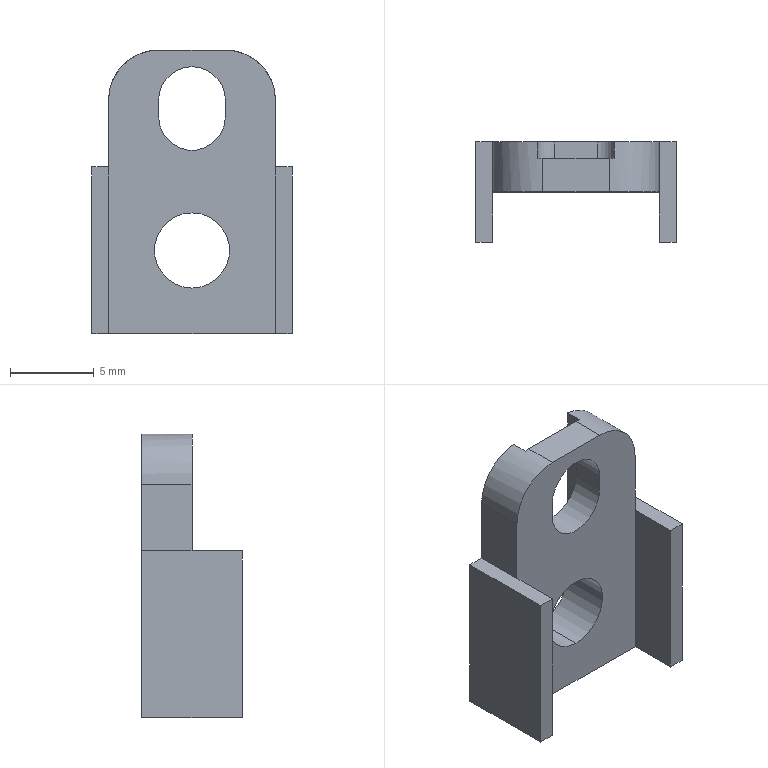Component | SolidWorks | BearingHousingAssembly-1_JawBuckleJaw2-1 | 1 solid | 29 faces | box 12 x 6 x 17 mm | volume 497 mm3 | plane 20 | cylinder 9 | commonest cylinder face diameters 4 x3 4.5 x2 6 x2 2 x2
build123d program:
from build123d import *

# Parameters (mm, degrees)
SKETCH1_W                  = 17
SKETCH1_H                  = 10
BOSS_EXTRUDE1_DEPTH        = 3
F_4_5_4_5_DIAMETER_HOLE1_D = 4.5
SKETCH4_W                  = 6
SKETCH4_H                  = 1
BOSS_EXTRUDE2_DEPTH        = 10
FILLET1_R                  = 3
CUT_EXTRUDE1_DEPTH         = 20
SKETCH6_W                  = 11.734
SKETCH6_H                  = 4.6
CUT_EXTRUDE2_DEPTH         = 1
FILLET2_R                  = 1


with BuildPart() as part:
    # Sketch1 → Boss-Extrude1 (new body)
    with BuildSketch(Plane.XY):
        with Locations((8.5, 0)):
            Rectangle(SKETCH1_W, SKETCH1_H)
    extrude(amount=BOSS_EXTRUDE1_DEPTH)

    # 4.5 _4.5_ Diameter Hole1 (through all)
    with Locations(Plane(origin=(0, 0, 0), x_dir=(-1, 0, 0), z_dir=(0, 0, -1))):
        with Locations((-5, 0)):
            Hole(F_4_5_4_5_DIAMETER_HOLE1_D / 2)

    # Sketch4 → Boss-Extrude2 (add)
    with BuildSketch(Plane.ZY):
        with Locations((0, 5.5)):
            Rectangle(SKETCH4_W, SKETCH4_H)
        with Locations((0, -5.5)):
            Rectangle(SKETCH4_W, SKETCH4_H)
    extrude(amount=-BOSS_EXTRUDE2_DEPTH)

    # Fillet1
    fillet1_edges = [part.edges().sort_by_distance(p)[0] for p in [
        (17, -5, 1.5),
        (17, 5, 1.5),
    ]]
    fillet(fillet1_edges, radius=FILLET1_R)

    # Sketch5 → Cut-Extrude1 (cut, through all)
    with BuildSketch(Plane.XY.offset(3)):
        with BuildLine():
            Line((13, 2), (14, 2))
            ThreePointArc((14, 2), (16, 0), (14, -2))
            Line((14, -2), (13, -2))
            ThreePointArc((13, -2), (11, 0), (13, 2))
        make_face()
    extrude(amount=-CUT_EXTRUDE1_DEPTH, mode=Mode.SUBTRACT)

    # Sketch6 → Cut-Extrude2 (cut)
    with BuildSketch(Plane.XY.offset(3)):
        with Locations((13.867, 0)):
            Rectangle(SKETCH6_W, SKETCH6_H)
    extrude(amount=-CUT_EXTRUDE2_DEPTH, mode=Mode.SUBTRACT)

    # Fillet2
    fillet2_edges = [part.edges().sort_by_distance(p)[0] for p in [
        (8, -2.3, 2.5),
        (8, 2.3, 2.5),
    ]]
    fillet(fillet2_edges, radius=FILLET2_R)


solid = part.part

# Placed as in the assembly
solid = solid.moved(Location((-38.666, 341.064, -6), (-90, 0, -90)))
STEP:
#1=CARTESIAN_POINT('',(-1.522,13.546,0.04921));
#2=VERTEX_POINT('',#1);
#3=CARTESIAN_POINT('',(-1.522,13.546,-0.128));
#4=VERTEX_POINT('',#3);
#5=CARTESIAN_POINT('',(-1.522,13.546,-0.03937));
#6=DIRECTION('',(-0.,-1.,0.));
#7=DIRECTION('',(-0.,0.,-1.));
#8=AXIS2_PLACEMENT_3D('',#5,#6,#7);
#9=CIRCLE('',#8,0.08858);
#10=EDGE_CURVE('',#2,#4,#9,.T.);
#11=ORIENTED_EDGE('',*,*,#10,.F.);
#12=CARTESIAN_POINT('',(-1.522,13.428,0.04921));
#13=VERTEX_POINT('',#12);
#14=CARTESIAN_POINT('',(-1.522,13.428,0.04921));
#15=DIRECTION('',(-0.,-1.,0.));
#16=VECTOR('',#15,39.37);
#17=LINE('',#14,#16);
#18=EDGE_CURVE('',#2,#13,#17,.T.);
#19=ORIENTED_EDGE('',*,*,#18,.T.);
#20=CARTESIAN_POINT('',(-1.522,13.428,-0.128));
#21=VERTEX_POINT('',#20);
#22=CARTESIAN_POINT('',(-1.522,13.428,-0.03937));
#23=DIRECTION('',(-0.,-1.,0.));
#24=DIRECTION('',(-0.,0.,-1.));
#25=AXIS2_PLACEMENT_3D('',#22,#23,#24);
#26=CIRCLE('',#25,0.08858);
#27=EDGE_CURVE('',#13,#21,#26,.T.);
#28=ORIENTED_EDGE('',*,*,#27,.T.);
#29=CARTESIAN_POINT('',(-1.522,13.428,-0.128));
#30=DIRECTION('',(-0.,-1.,0.));
#31=VECTOR('',#30,39.37);
#32=LINE('',#29,#31);
#33=EDGE_CURVE('',#4,#21,#32,.T.);
#34=ORIENTED_EDGE('',*,*,#33,.F.);
#35=EDGE_LOOP('',(#11,#19,#28,#34));
#36=FACE_OUTER_BOUND('',#35,.T.);
#37=CARTESIAN_POINT('',(-1.522,13.428,-0.03937));
#38=DIRECTION('',(-0.,-1.,0.));
#39=DIRECTION('',(-0.,0.,-1.));
#40=AXIS2_PLACEMENT_3D('',#37,#38,#39);
#41=CYLINDRICAL_SURFACE('',#40,0.08858);
#42=ADVANCED_FACE('',(#36),#41,.F.);
#43=CARTESIAN_POINT('',(-1.522,13.428,0.3937));
#44=VERTEX_POINT('',#43);
#45=CARTESIAN_POINT('',(-1.444,13.428,0.315));
#46=VERTEX_POINT('',#45);
#47=CARTESIAN_POINT('',(-1.522,13.428,0.315));
#48=DIRECTION('',(0.,1.,-0.));
#49=DIRECTION('',(0.,0.,1.));
#50=AXIS2_PLACEMENT_3D('',#47,#48,#49);
#51=CIRCLE('',#50,0.07874);
#52=EDGE_CURVE('',#44,#46,#51,.T.);
#53=ORIENTED_EDGE('',*,*,#52,.F.);
#54=CARTESIAN_POINT('',(-1.522,13.506,0.3937));
#55=VERTEX_POINT('',#54);
#56=CARTESIAN_POINT('',(-1.522,13.31,0.3937));
#57=DIRECTION('',(0.,1.,-0.));
#58=VECTOR('',#57,39.37);
#59=LINE('',#56,#58);
#60=EDGE_CURVE('',#44,#55,#59,.T.);
#61=ORIENTED_EDGE('',*,*,#60,.T.);
#62=CARTESIAN_POINT('',(-1.444,13.506,0.315));
#63=VERTEX_POINT('',#62);
#64=CARTESIAN_POINT('',(-1.522,13.506,0.315));
#65=DIRECTION('',(-0.,-1.,0.));
#66=DIRECTION('',(0.,0.,1.));
#67=AXIS2_PLACEMENT_3D('',#64,#65,#66);
#68=CIRCLE('',#67,0.07874);
#69=EDGE_CURVE('',#63,#55,#68,.T.);
#70=ORIENTED_EDGE('',*,*,#69,.F.);
#71=CARTESIAN_POINT('',(-1.444,13.31,0.315));
#72=DIRECTION('',(0.,1.,-0.));
#73=VECTOR('',#72,39.37);
#74=LINE('',#71,#73);
#75=EDGE_CURVE('',#46,#63,#74,.T.);
#76=ORIENTED_EDGE('',*,*,#75,.F.);
#77=EDGE_LOOP('',(#53,#61,#70,#76));
#78=FACE_OUTER_BOUND('',#77,.T.);
#79=CARTESIAN_POINT('',(-1.522,13.31,0.315));
#80=DIRECTION('',(0.,1.,-0.));
#81=DIRECTION('',(0.,0.,1.));
#82=AXIS2_PLACEMENT_3D('',#79,#80,#81);
#83=CYLINDRICAL_SURFACE('',#82,0.07874);
#84=ADVANCED_FACE('',(#78),#83,.F.);
#85=CARTESIAN_POINT('',(-1.601,13.506,0.4331));
#86=VERTEX_POINT('',#85);
#87=CARTESIAN_POINT('',(-1.444,13.506,0.4331));
#88=VERTEX_POINT('',#87);
#89=CARTESIAN_POINT('',(-1.325,13.506,0.4331));
#90=DIRECTION('',(1.,-0.,-0.));
#91=VECTOR('',#90,39.37);
#92=LINE('',#89,#91);
#93=EDGE_CURVE('',#86,#88,#92,.T.);
#94=ORIENTED_EDGE('',*,*,#93,.F.);
#95=CARTESIAN_POINT('',(-1.601,13.428,0.4331));
#96=VERTEX_POINT('',#95);
#97=CARTESIAN_POINT('',(-1.601,13.546,0.4331));
#98=DIRECTION('',(-0.,-1.,0.));
#99=VECTOR('',#98,39.37);
#100=LINE('',#97,#99);
#101=EDGE_CURVE('',#86,#96,#100,.T.);
#102=ORIENTED_EDGE('',*,*,#101,.T.);
#103=CARTESIAN_POINT('',(-1.444,13.428,0.4331));
#104=VERTEX_POINT('',#103);
#105=CARTESIAN_POINT('',(-1.325,13.428,0.4331));
#106=DIRECTION('',(1.,-0.,-0.));
#107=VECTOR('',#106,39.37);
#108=LINE('',#105,#107);
#109=EDGE_CURVE('',#96,#104,#108,.T.);
#110=ORIENTED_EDGE('',*,*,#109,.T.);
#111=CARTESIAN_POINT('',(-1.444,13.546,0.4331));
#112=DIRECTION('',(0.,1.,-0.));
#113=VECTOR('',#112,39.37);
#114=LINE('',#111,#113);
#115=EDGE_CURVE('',#104,#88,#114,.T.);
#116=ORIENTED_EDGE('',*,*,#115,.T.);
#117=EDGE_LOOP('',(#94,#102,#110,#116));
#118=FACE_OUTER_BOUND('',#117,.T.);
#119=CARTESIAN_POINT('',(-1.325,13.546,0.4331));
#120=DIRECTION('',(-0.,-0.,-1.));
#121=DIRECTION('',(0.,1.,-0.));
#122=AXIS2_PLACEMENT_3D('',#119,#120,#121);
#123=PLANE('',#122);
#124=ADVANCED_FACE('',(#118),#123,.F.);
#125=CARTESIAN_POINT('',(-1.601,13.506,0.2756));
#126=VERTEX_POINT('',#125);
#127=CARTESIAN_POINT('',(-1.444,13.506,0.2756));
#128=VERTEX_POINT('',#127);
#129=CARTESIAN_POINT('',(-1.522,13.506,0.2756));
#130=DIRECTION('',(-0.,-1.,0.));
#131=DIRECTION('',(0.,0.,1.));
#132=AXIS2_PLACEMENT_3D('',#129,#130,#131);
#133=CIRCLE('',#132,0.07874);
#134=EDGE_CURVE('',#126,#128,#133,.T.);
#135=ORIENTED_EDGE('',*,*,#134,.F.);
#136=CARTESIAN_POINT('',(-1.601,13.428,0.2756));
#137=VERTEX_POINT('',#136);
#138=CARTESIAN_POINT('',(-1.601,13.31,0.2756));
#139=DIRECTION('',(0.,1.,-0.));
#140=VECTOR('',#139,39.37);
#141=LINE('',#138,#140);
#142=EDGE_CURVE('',#137,#126,#141,.T.);
#143=ORIENTED_EDGE('',*,*,#142,.F.);
#144=CARTESIAN_POINT('',(-1.444,13.428,0.2756));
#145=VERTEX_POINT('',#144);
#146=CARTESIAN_POINT('',(-1.522,13.428,0.2756));
#147=DIRECTION('',(0.,1.,-0.));
#148=DIRECTION('',(0.,0.,1.));
#149=AXIS2_PLACEMENT_3D('',#146,#147,#148);
#150=CIRCLE('',#149,0.07874);
#151=EDGE_CURVE('',#145,#137,#150,.T.);
#152=ORIENTED_EDGE('',*,*,#151,.F.);
#153=CARTESIAN_POINT('',(-1.444,13.31,0.2756));
#154=DIRECTION('',(0.,1.,-0.));
#155=VECTOR('',#154,39.37);
#156=LINE('',#153,#155);
#157=EDGE_CURVE('',#145,#128,#156,.T.);
#158=ORIENTED_EDGE('',*,*,#157,.T.);
#159=EDGE_LOOP('',(#135,#143,#152,#158));
#160=FACE_OUTER_BOUND('',#159,.T.);
#161=CARTESIAN_POINT('',(-1.522,13.31,0.2756));
#162=DIRECTION('',(0.,1.,-0.));
#163=DIRECTION('',(0.,0.,1.));
#164=AXIS2_PLACEMENT_3D('',#161,#162,#163);
#165=CYLINDRICAL_SURFACE('',#164,0.07874);
#166=ADVANCED_FACE('',(#160),#165,.F.);
#167=CARTESIAN_POINT('',(-1.444,13.506,0.2756));
#168=DIRECTION('',(0.,0.,1.));
#169=VECTOR('',#168,39.37);
#170=LINE('',#167,#169);
#171=EDGE_CURVE('',#128,#63,#170,.T.);
#172=ORIENTED_EDGE('',*,*,#171,.F.);
#173=ORIENTED_EDGE('',*,*,#157,.F.);
#174=CARTESIAN_POINT('',(-1.444,13.428,-0.2362));
#175=DIRECTION('',(-0.,-0.,-1.));
#176=VECTOR('',#175,39.37);
#177=LINE('',#174,#176);
#178=EDGE_CURVE('',#46,#145,#177,.T.);
#179=ORIENTED_EDGE('',*,*,#178,.F.);
#180=ORIENTED_EDGE('',*,*,#75,.T.);
#181=EDGE_LOOP('',(#172,#173,#179,#180));
#182=FACE_OUTER_BOUND('',#181,.T.);
#183=CARTESIAN_POINT('',(-1.444,13.31,0.2756));
#184=DIRECTION('',(1.,-0.,-0.));
#185=DIRECTION('',(0.,1.,-0.));
#186=AXIS2_PLACEMENT_3D('',#183,#184,#185);
#187=PLANE('',#186);
#188=ADVANCED_FACE('',(#182),#187,.F.);
#189=ORIENTED_EDGE('',*,*,#60,.F.);
#190=CARTESIAN_POINT('',(-1.601,13.428,0.315));
#191=VERTEX_POINT('',#190);
#192=CARTESIAN_POINT('',(-1.522,13.428,0.315));
#193=DIRECTION('',(0.,1.,-0.));
#194=DIRECTION('',(0.,0.,1.));
#195=AXIS2_PLACEMENT_3D('',#192,#193,#194);
#196=CIRCLE('',#195,0.07874);
#197=EDGE_CURVE('',#191,#44,#196,.T.);
#198=ORIENTED_EDGE('',*,*,#197,.F.);
#199=CARTESIAN_POINT('',(-1.601,13.506,0.315));
#200=VERTEX_POINT('',#199);
#201=CARTESIAN_POINT('',(-1.601,13.31,0.315));
#202=DIRECTION('',(0.,1.,-0.));
#203=VECTOR('',#202,39.37);
#204=LINE('',#201,#203);
#205=EDGE_CURVE('',#191,#200,#204,.T.);
#206=ORIENTED_EDGE('',*,*,#205,.T.);
#207=CARTESIAN_POINT('',(-1.522,13.506,0.315));
#208=DIRECTION('',(-0.,-1.,0.));
#209=DIRECTION('',(0.,0.,1.));
#210=AXIS2_PLACEMENT_3D('',#207,#208,#209);
#211=CIRCLE('',#210,0.07874);
#212=EDGE_CURVE('',#55,#200,#211,.T.);
#213=ORIENTED_EDGE('',*,*,#212,.F.);
#214=EDGE_LOOP('',(#189,#198,#206,#213));
#215=FACE_OUTER_BOUND('',#214,.T.);
#216=CARTESIAN_POINT('',(-1.522,13.31,0.315));
#217=DIRECTION('',(0.,1.,-0.));
#218=DIRECTION('',(0.,0.,1.));
#219=AXIS2_PLACEMENT_3D('',#216,#217,#218);
#220=CYLINDRICAL_SURFACE('',#219,0.07874);
#221=ADVANCED_FACE('',(#215),#220,.F.);
#222=CARTESIAN_POINT('',(-1.601,13.506,0.2756));
#223=DIRECTION('',(-0.,-0.,-1.));
#224=VECTOR('',#223,39.37);
#225=LINE('',#222,#224);
#226=EDGE_CURVE('',#200,#126,#225,.T.);
#227=ORIENTED_EDGE('',*,*,#226,.F.);
#228=ORIENTED_EDGE('',*,*,#205,.F.);
#229=CARTESIAN_POINT('',(-1.601,13.428,-0.2362));
#230=DIRECTION('',(0.,0.,1.));
#231=VECTOR('',#230,39.37);
#232=LINE('',#229,#231);
#233=EDGE_CURVE('',#137,#191,#232,.T.);
#234=ORIENTED_EDGE('',*,*,#233,.F.);
#235=ORIENTED_EDGE('',*,*,#142,.T.);
#236=EDGE_LOOP('',(#227,#228,#234,#235));
#237=FACE_OUTER_BOUND('',#236,.T.);
#238=CARTESIAN_POINT('',(-1.601,13.31,0.2756));
#239=DIRECTION('',(-1.,0.,0.));
#240=DIRECTION('',(-0.,-1.,0.));
#241=AXIS2_PLACEMENT_3D('',#238,#239,#240);
#242=PLANE('',#241);
#243=ADVANCED_FACE('',(#237),#242,.F.);
#244=CARTESIAN_POINT('',(-1.325,13.428,-0.2362));
#245=VERTEX_POINT('',#244);
#246=CARTESIAN_POINT('',(-1.719,13.428,-0.2362));
#247=VERTEX_POINT('',#246);
#248=CARTESIAN_POINT('',(-1.325,13.428,-0.2362));
#249=DIRECTION('',(-1.,0.,0.));
#250=VECTOR('',#249,39.37);
#251=LINE('',#248,#250);
#252=EDGE_CURVE('',#245,#247,#251,.T.);
#253=ORIENTED_EDGE('',*,*,#252,.T.);
#254=CARTESIAN_POINT('',(-1.719,13.31,-0.2362));
#255=VERTEX_POINT('',#254);
#256=CARTESIAN_POINT('',(-1.719,13.546,-0.2362));
#257=DIRECTION('',(-0.,-1.,0.));
#258=VECTOR('',#257,39.37);
#259=LINE('',#256,#258);
#260=EDGE_CURVE('',#247,#255,#259,.T.);
#261=ORIENTED_EDGE('',*,*,#260,.T.);
#262=CARTESIAN_POINT('',(-1.758,13.31,-0.2362));
#263=VERTEX_POINT('',#262);
#264=CARTESIAN_POINT('',(-1.719,13.31,-0.2362));
#265=DIRECTION('',(-1.,0.,0.));
#266=VECTOR('',#265,39.37);
#267=LINE('',#264,#266);
#268=EDGE_CURVE('',#255,#263,#267,.T.);
#269=ORIENTED_EDGE('',*,*,#268,.T.);
#270=CARTESIAN_POINT('',(-1.758,13.546,-0.2362));
#271=VERTEX_POINT('',#270);
#272=CARTESIAN_POINT('',(-1.758,13.546,-0.2362));
#273=DIRECTION('',(0.,1.,-0.));
#274=VECTOR('',#273,39.37);
#275=LINE('',#272,#274);
#276=EDGE_CURVE('',#263,#271,#275,.T.);
#277=ORIENTED_EDGE('',*,*,#276,.T.);
#278=CARTESIAN_POINT('',(-1.286,13.546,-0.2362));
#279=VERTEX_POINT('',#278);
#280=CARTESIAN_POINT('',(-1.325,13.546,-0.2362));
#281=DIRECTION('',(-1.,0.,0.));
#282=VECTOR('',#281,39.37);
#283=LINE('',#280,#282);
#284=EDGE_CURVE('',#279,#271,#283,.T.);
#285=ORIENTED_EDGE('',*,*,#284,.F.);
#286=CARTESIAN_POINT('',(-1.286,13.31,-0.2362));
#287=VERTEX_POINT('',#286);
#288=CARTESIAN_POINT('',(-1.286,13.546,-0.2362));
#289=DIRECTION('',(-0.,-1.,0.));
#290=VECTOR('',#289,39.37);
#291=LINE('',#288,#290);
#292=EDGE_CURVE('',#279,#287,#291,.T.);
#293=ORIENTED_EDGE('',*,*,#292,.T.);
#294=CARTESIAN_POINT('',(-1.325,13.31,-0.2362));
#295=VERTEX_POINT('',#294);
#296=CARTESIAN_POINT('',(-1.325,13.31,-0.2362));
#297=DIRECTION('',(-1.,0.,0.));
#298=VECTOR('',#297,39.37);
#299=LINE('',#296,#298);
#300=EDGE_CURVE('',#287,#295,#299,.T.);
#301=ORIENTED_EDGE('',*,*,#300,.T.);
#302=CARTESIAN_POINT('',(-1.325,13.546,-0.2362));
#303=DIRECTION('',(0.,1.,-0.));
#304=VECTOR('',#303,39.37);
#305=LINE('',#302,#304);
#306=EDGE_CURVE('',#295,#245,#305,.T.);
#307=ORIENTED_EDGE('',*,*,#306,.T.);
#308=EDGE_LOOP('',(#253,#261,#269,#277,#285,#293,#301,#307));
#309=FACE_OUTER_BOUND('',#308,.T.);
#310=CARTESIAN_POINT('',(-1.325,13.546,-0.2362));
#311=DIRECTION('',(0.,0.,1.));
#312=DIRECTION('',(1.,-0.,-0.));
#313=AXIS2_PLACEMENT_3D('',#310,#311,#312);
#314=PLANE('',#313);
#315=ADVANCED_FACE('',(#309),#314,.F.);
#316=CARTESIAN_POINT('',(-1.719,13.428,0.1575));
#317=VERTEX_POINT('',#316);
#318=CARTESIAN_POINT('',(-1.719,13.428,0.315));
#319=VERTEX_POINT('',#318);
#320=CARTESIAN_POINT('',(-1.719,13.428,-0.2362));
#321=DIRECTION('',(0.,0.,1.));
#322=VECTOR('',#321,39.37);
#323=LINE('',#320,#322);
#324=EDGE_CURVE('',#317,#319,#323,.T.);
#325=ORIENTED_EDGE('',*,*,#324,.T.);
#326=CARTESIAN_POINT('',(-1.719,13.546,0.315));
#327=VERTEX_POINT('',#326);
#328=CARTESIAN_POINT('',(-1.719,13.546,0.315));
#329=DIRECTION('',(0.,1.,-0.));
#330=VECTOR('',#329,39.37);
#331=LINE('',#328,#330);
#332=EDGE_CURVE('',#319,#327,#331,.T.);
#333=ORIENTED_EDGE('',*,*,#332,.T.);
#334=CARTESIAN_POINT('',(-1.719,13.546,0.1575));
#335=VERTEX_POINT('',#334);
#336=CARTESIAN_POINT('',(-1.719,13.546,-0.2362));
#337=DIRECTION('',(0.,0.,1.));
#338=VECTOR('',#337,39.37);
#339=LINE('',#336,#338);
#340=EDGE_CURVE('',#335,#327,#339,.T.);
#341=ORIENTED_EDGE('',*,*,#340,.F.);
#342=CARTESIAN_POINT('',(-1.719,13.546,0.1575));
#343=DIRECTION('',(-0.,-1.,0.));
#344=VECTOR('',#343,39.37);
#345=LINE('',#342,#344);
#346=EDGE_CURVE('',#335,#317,#345,.T.);
#347=ORIENTED_EDGE('',*,*,#346,.T.);
#348=EDGE_LOOP('',(#325,#333,#341,#347));
#349=FACE_OUTER_BOUND('',#348,.T.);
#350=CARTESIAN_POINT('',(-1.719,13.546,-0.2362));
#351=DIRECTION('',(1.,-0.,-0.));
#352=DIRECTION('',(0.,1.,-0.));
#353=AXIS2_PLACEMENT_3D('',#350,#351,#352);
#354=PLANE('',#353);
#355=ADVANCED_FACE('',(#349),#354,.F.);
#356=CARTESIAN_POINT('',(-1.325,13.546,0.315));
#357=VERTEX_POINT('',#356);
#358=CARTESIAN_POINT('',(-1.325,13.546,0.1575));
#359=VERTEX_POINT('',#358);
#360=CARTESIAN_POINT('',(-1.325,13.546,-0.2362));
#361=DIRECTION('',(-0.,-0.,-1.));
#362=VECTOR('',#361,39.37);
#363=LINE('',#360,#362);
#364=EDGE_CURVE('',#357,#359,#363,.T.);
#365=ORIENTED_EDGE('',*,*,#364,.F.);
#366=CARTESIAN_POINT('',(-1.325,13.428,0.315));
#367=VERTEX_POINT('',#366);
#368=CARTESIAN_POINT('',(-1.325,13.546,0.315));
#369=DIRECTION('',(-0.,-1.,0.));
#370=VECTOR('',#369,39.37);
#371=LINE('',#368,#370);
#372=EDGE_CURVE('',#357,#367,#371,.T.);
#373=ORIENTED_EDGE('',*,*,#372,.T.);
#374=CARTESIAN_POINT('',(-1.325,13.428,0.1575));
#375=VERTEX_POINT('',#374);
#376=CARTESIAN_POINT('',(-1.325,13.428,-0.2362));
#377=DIRECTION('',(-0.,-0.,-1.));
#378=VECTOR('',#377,39.37);
#379=LINE('',#376,#378);
#380=EDGE_CURVE('',#367,#375,#379,.T.);
#381=ORIENTED_EDGE('',*,*,#380,.T.);
#382=CARTESIAN_POINT('',(-1.325,13.546,0.1575));
#383=DIRECTION('',(0.,1.,-0.));
#384=VECTOR('',#383,39.37);
#385=LINE('',#382,#384);
#386=EDGE_CURVE('',#375,#359,#385,.T.);
#387=ORIENTED_EDGE('',*,*,#386,.T.);
#388=EDGE_LOOP('',(#365,#373,#381,#387));
#389=FACE_OUTER_BOUND('',#388,.T.);
#390=CARTESIAN_POINT('',(-1.325,13.546,-0.2362));
#391=DIRECTION('',(-1.,0.,0.));
#392=DIRECTION('',(-0.,-1.,0.));
#393=AXIS2_PLACEMENT_3D('',#390,#391,#392);
#394=PLANE('',#393);
#395=ADVANCED_FACE('',(#389),#394,.F.);
#396=CARTESIAN_POINT('',(-1.432,13.546,0.4325));
#397=VERTEX_POINT('',#396);
#398=CARTESIAN_POINT('',(-1.432,13.546,0.1181));
#399=VERTEX_POINT('',#398);
#400=CARTESIAN_POINT('',(-1.432,13.546,0.07874));
#401=DIRECTION('',(-0.,-0.,-1.));
#402=VECTOR('',#401,39.37);
#403=LINE('',#400,#402);
#404=EDGE_CURVE('',#397,#399,#403,.T.);
#405=ORIENTED_EDGE('',*,*,#404,.F.);
#406=CARTESIAN_POINT('',(-1.444,13.546,0.315));
#407=DIRECTION('',(0.,1.,-0.));
#408=DIRECTION('',(0.,0.,1.));
#409=AXIS2_PLACEMENT_3D('',#406,#407,#408);
#410=CIRCLE('',#409,0.1181);
#411=EDGE_CURVE('',#397,#357,#410,.T.);
#412=ORIENTED_EDGE('',*,*,#411,.T.);
#413=ORIENTED_EDGE('',*,*,#364,.T.);
#414=CARTESIAN_POINT('',(-1.286,13.546,0.1575));
#415=VERTEX_POINT('',#414);
#416=CARTESIAN_POINT('',(-1.325,13.546,0.1575));
#417=DIRECTION('',(1.,-0.,-0.));
#418=VECTOR('',#417,39.37);
#419=LINE('',#416,#418);
#420=EDGE_CURVE('',#359,#415,#419,.T.);
#421=ORIENTED_EDGE('',*,*,#420,.T.);
#422=CARTESIAN_POINT('',(-1.286,13.546,0.1575));
#423=DIRECTION('',(-0.,-0.,-1.));
#424=VECTOR('',#423,39.37);
#425=LINE('',#422,#424);
#426=EDGE_CURVE('',#415,#279,#425,.T.);
#427=ORIENTED_EDGE('',*,*,#426,.T.);
#428=ORIENTED_EDGE('',*,*,#284,.T.);
#429=CARTESIAN_POINT('',(-1.758,13.546,0.1575));
#430=VERTEX_POINT('',#429);
#431=CARTESIAN_POINT('',(-1.758,13.546,0.1575));
#432=DIRECTION('',(-0.,-0.,-1.));
#433=VECTOR('',#432,39.37);
#434=LINE('',#431,#433);
#435=EDGE_CURVE('',#430,#271,#434,.T.);
#436=ORIENTED_EDGE('',*,*,#435,.F.);
#437=CARTESIAN_POINT('',(-1.719,13.546,0.1575));
#438=DIRECTION('',(1.,0.,-0.));
#439=VECTOR('',#438,39.37);
#440=LINE('',#437,#439);
#441=EDGE_CURVE('',#430,#335,#440,.T.);
#442=ORIENTED_EDGE('',*,*,#441,.T.);
#443=ORIENTED_EDGE('',*,*,#340,.T.);
#444=CARTESIAN_POINT('',(-1.613,13.546,0.4325));
#445=VERTEX_POINT('',#444);
#446=CARTESIAN_POINT('',(-1.601,13.546,0.315));
#447=DIRECTION('',(0.,1.,-0.));
#448=DIRECTION('',(0.,0.,1.));
#449=AXIS2_PLACEMENT_3D('',#446,#447,#448);
#450=CIRCLE('',#449,0.1181);
#451=EDGE_CURVE('',#327,#445,#450,.T.);
#452=ORIENTED_EDGE('',*,*,#451,.T.);
#453=CARTESIAN_POINT('',(-1.613,13.546,0.1181));
#454=VERTEX_POINT('',#453);
#455=CARTESIAN_POINT('',(-1.613,13.546,0.07874));
#456=DIRECTION('',(0.,0.,1.));
#457=VECTOR('',#456,39.37);
#458=LINE('',#455,#457);
#459=EDGE_CURVE('',#454,#445,#458,.T.);
#460=ORIENTED_EDGE('',*,*,#459,.F.);
#461=CARTESIAN_POINT('',(-1.573,13.546,0.07874));
#462=VERTEX_POINT('',#461);
#463=CARTESIAN_POINT('',(-1.573,13.546,0.1181));
#464=DIRECTION('',(-0.,-1.,0.));
#465=DIRECTION('',(0.,0.,1.));
#466=AXIS2_PLACEMENT_3D('',#463,#464,#465);
#467=CIRCLE('',#466,0.03937);
#468=EDGE_CURVE('',#454,#462,#467,.T.);
#469=ORIENTED_EDGE('',*,*,#468,.T.);
#470=CARTESIAN_POINT('',(-1.471,13.546,0.07874));
#471=VERTEX_POINT('',#470);
#472=CARTESIAN_POINT('',(-1.432,13.546,0.07874));
#473=DIRECTION('',(-1.,0.,0.));
#474=VECTOR('',#473,39.37);
#475=LINE('',#472,#474);
#476=EDGE_CURVE('',#471,#462,#475,.T.);
#477=ORIENTED_EDGE('',*,*,#476,.F.);
#478=CARTESIAN_POINT('',(-1.471,13.546,0.1181));
#479=DIRECTION('',(-0.,-1.,0.));
#480=DIRECTION('',(0.,0.,1.));
#481=AXIS2_PLACEMENT_3D('',#478,#479,#480);
#482=CIRCLE('',#481,0.03937);
#483=EDGE_CURVE('',#471,#399,#482,.T.);
#484=ORIENTED_EDGE('',*,*,#483,.T.);
#485=EDGE_LOOP('',(#405,#412,#413,#421,#427,#428,#436,#442,#443,#452,#460,#469,#477,#484));
#486=FACE_OUTER_BOUND('',#485,.T.);
#487=CARTESIAN_POINT('',(-1.522,13.546,-0.03937));
#488=DIRECTION('',(-0.,-1.,0.));
#489=DIRECTION('',(-0.,0.,-1.));
#490=AXIS2_PLACEMENT_3D('',#487,#488,#489);
#491=CIRCLE('',#490,0.08858);
#492=EDGE_CURVE('',#4,#2,#491,.T.);
#493=ORIENTED_EDGE('',*,*,#492,.T.);
#494=ORIENTED_EDGE('',*,*,#10,.T.);
#495=EDGE_LOOP('',(#493,#494));
#496=FACE_BOUND('',#495,.T.);
#497=CARTESIAN_POINT('',(-1.522,13.546,-0.2362));
#498=DIRECTION('',(0.,1.,-0.));
#499=DIRECTION('',(0.,0.,1.));
#500=AXIS2_PLACEMENT_3D('',#497,#498,#499);
#501=PLANE('',#500);
#502=ADVANCED_FACE('',(#486,#496),#501,.T.);
#503=ORIENTED_EDGE('',*,*,#178,.T.);
#504=ORIENTED_EDGE('',*,*,#151,.T.);
#505=ORIENTED_EDGE('',*,*,#233,.T.);
#506=ORIENTED_EDGE('',*,*,#197,.T.);
#507=ORIENTED_EDGE('',*,*,#52,.T.);
#508=EDGE_LOOP('',(#503,#504,#505,#506,#507));
#509=FACE_BOUND('',#508,.T.);
#510=CARTESIAN_POINT('',(-1.522,13.428,-0.03937));
#511=DIRECTION('',(-0.,-1.,0.));
#512=DIRECTION('',(-0.,0.,-1.));
#513=AXIS2_PLACEMENT_3D('',#510,#511,#512);
#514=CIRCLE('',#513,0.08858);
#515=EDGE_CURVE('',#21,#13,#514,.T.);
#516=ORIENTED_EDGE('',*,*,#515,.F.);
#517=ORIENTED_EDGE('',*,*,#27,.F.);
#518=EDGE_LOOP('',(#516,#517));
#519=FACE_BOUND('',#518,.T.);
#520=ORIENTED_EDGE('',*,*,#109,.F.);
#521=CARTESIAN_POINT('',(-1.601,13.428,0.315));
#522=DIRECTION('',(-0.,-1.,0.));
#523=DIRECTION('',(0.,0.,1.));
#524=AXIS2_PLACEMENT_3D('',#521,#522,#523);
#525=CIRCLE('',#524,0.1181);
#526=EDGE_CURVE('',#96,#319,#525,.T.);
#527=ORIENTED_EDGE('',*,*,#526,.T.);
#528=ORIENTED_EDGE('',*,*,#324,.F.);
#529=CARTESIAN_POINT('',(-1.719,13.428,-0.2362));
#530=DIRECTION('',(0.,0.,1.));
#531=VECTOR('',#530,39.37);
#532=LINE('',#529,#531);
#533=EDGE_CURVE('',#247,#317,#532,.T.);
#534=ORIENTED_EDGE('',*,*,#533,.F.);
#535=ORIENTED_EDGE('',*,*,#252,.F.);
#536=CARTESIAN_POINT('',(-1.325,13.428,-0.2362));
#537=DIRECTION('',(-0.,-0.,-1.));
#538=VECTOR('',#537,39.37);
#539=LINE('',#536,#538);
#540=EDGE_CURVE('',#375,#245,#539,.T.);
#541=ORIENTED_EDGE('',*,*,#540,.F.);
#542=ORIENTED_EDGE('',*,*,#380,.F.);
#543=CARTESIAN_POINT('',(-1.444,13.428,0.315));
#544=DIRECTION('',(-0.,-1.,0.));
#545=DIRECTION('',(0.,0.,1.));
#546=AXIS2_PLACEMENT_3D('',#543,#544,#545);
#547=CIRCLE('',#546,0.1181);
#548=EDGE_CURVE('',#367,#104,#547,.T.);
#549=ORIENTED_EDGE('',*,*,#548,.T.);
#550=EDGE_LOOP('',(#520,#527,#528,#534,#535,#541,#542,#549));
#551=FACE_OUTER_BOUND('',#550,.T.);
#552=CARTESIAN_POINT('',(-1.522,13.428,-0.2362));
#553=DIRECTION('',(0.,1.,-0.));
#554=DIRECTION('',(0.,0.,1.));
#555=AXIS2_PLACEMENT_3D('',#552,#553,#554);
#556=PLANE('',#555);
#557=ADVANCED_FACE('',(#509,#519,#551),#556,.F.);
#558=ORIENTED_EDGE('',*,*,#18,.F.);
#559=ORIENTED_EDGE('',*,*,#492,.F.);
#560=ORIENTED_EDGE('',*,*,#33,.T.);
#561=ORIENTED_EDGE('',*,*,#515,.T.);
#562=EDGE_LOOP('',(#558,#559,#560,#561));
#563=FACE_OUTER_BOUND('',#562,.T.);
#564=CARTESIAN_POINT('',(-1.522,13.428,-0.03937));
#565=DIRECTION('',(-0.,-1.,0.));
#566=DIRECTION('',(-0.,0.,-1.));
#567=AXIS2_PLACEMENT_3D('',#564,#565,#566);
#568=CYLINDRICAL_SURFACE('',#567,0.08858);
#569=ADVANCED_FACE('',(#563),#568,.F.);
#570=CARTESIAN_POINT('',(-1.325,13.31,0.1575));
#571=VERTEX_POINT('',#570);
#572=CARTESIAN_POINT('',(-1.325,13.546,0.1575));
#573=DIRECTION('',(0.,1.,-0.));
#574=VECTOR('',#573,39.37);
#575=LINE('',#572,#574);
#576=EDGE_CURVE('',#571,#375,#575,.T.);
#577=ORIENTED_EDGE('',*,*,#576,.T.);
#578=ORIENTED_EDGE('',*,*,#540,.T.);
#579=ORIENTED_EDGE('',*,*,#306,.F.);
#580=CARTESIAN_POINT('',(-1.325,13.31,0.1575));
#581=DIRECTION('',(-0.,-0.,-1.));
#582=VECTOR('',#581,39.37);
#583=LINE('',#580,#582);
#584=EDGE_CURVE('',#571,#295,#583,.T.);
#585=ORIENTED_EDGE('',*,*,#584,.F.);
#586=EDGE_LOOP('',(#577,#578,#579,#585));
#587=FACE_OUTER_BOUND('',#586,.T.);
#588=CARTESIAN_POINT('',(-1.325,13.546,0.1575));
#589=DIRECTION('',(-1.,0.,0.));
#590=DIRECTION('',(-0.,-1.,0.));
#591=AXIS2_PLACEMENT_3D('',#588,#589,#590);
#592=PLANE('',#591);
#593=ADVANCED_FACE('',(#587),#592,.T.);
#594=ORIENTED_EDGE('',*,*,#300,.F.);
#595=CARTESIAN_POINT('',(-1.286,13.31,0.1575));
#596=VERTEX_POINT('',#595);
#597=CARTESIAN_POINT('',(-1.286,13.31,0.1575));
#598=DIRECTION('',(-0.,-0.,-1.));
#599=VECTOR('',#598,39.37);
#600=LINE('',#597,#599);
#601=EDGE_CURVE('',#596,#287,#600,.T.);
#602=ORIENTED_EDGE('',*,*,#601,.F.);
#603=CARTESIAN_POINT('',(-1.325,13.31,0.1575));
#604=DIRECTION('',(-1.,0.,0.));
#605=VECTOR('',#604,39.37);
#606=LINE('',#603,#605);
#607=EDGE_CURVE('',#596,#571,#606,.T.);
#608=ORIENTED_EDGE('',*,*,#607,.T.);
#609=ORIENTED_EDGE('',*,*,#584,.T.);
#610=EDGE_LOOP('',(#594,#602,#608,#609));
#611=FACE_OUTER_BOUND('',#610,.T.);
#612=CARTESIAN_POINT('',(-1.325,13.31,0.1575));
#613=DIRECTION('',(-0.,-1.,0.));
#614=DIRECTION('',(-0.,-0.,-1.));
#615=AXIS2_PLACEMENT_3D('',#612,#613,#614);
#616=PLANE('',#615);
#617=ADVANCED_FACE('',(#611),#616,.T.);
#618=ORIENTED_EDGE('',*,*,#292,.F.);
#619=ORIENTED_EDGE('',*,*,#426,.F.);
#620=CARTESIAN_POINT('',(-1.286,13.546,0.1575));
#621=DIRECTION('',(-0.,-1.,0.));
#622=VECTOR('',#621,39.37);
#623=LINE('',#620,#622);
#624=EDGE_CURVE('',#415,#596,#623,.T.);
#625=ORIENTED_EDGE('',*,*,#624,.T.);
#626=ORIENTED_EDGE('',*,*,#601,.T.);
#627=EDGE_LOOP('',(#618,#619,#625,#626));
#628=FACE_OUTER_BOUND('',#627,.T.);
#629=CARTESIAN_POINT('',(-1.286,13.546,0.1575));
#630=DIRECTION('',(1.,-0.,-0.));
#631=DIRECTION('',(0.,1.,-0.));
#632=AXIS2_PLACEMENT_3D('',#629,#630,#631);
#633=PLANE('',#632);
#634=ADVANCED_FACE('',(#628),#633,.T.);
#635=ORIENTED_EDGE('',*,*,#420,.F.);
#636=ORIENTED_EDGE('',*,*,#386,.F.);
#637=ORIENTED_EDGE('',*,*,#576,.F.);
#638=ORIENTED_EDGE('',*,*,#607,.F.);
#639=ORIENTED_EDGE('',*,*,#624,.F.);
#640=EDGE_LOOP('',(#635,#636,#637,#638,#639));
#641=FACE_OUTER_BOUND('',#640,.T.);
#642=CARTESIAN_POINT('',(-1.522,13.428,0.1575));
#643=DIRECTION('',(-0.,-0.,-1.));
#644=DIRECTION('',(-1.,0.,0.));
#645=AXIS2_PLACEMENT_3D('',#642,#643,#644);
#646=PLANE('',#645);
#647=ADVANCED_FACE('',(#641),#646,.F.);
#648=ORIENTED_EDGE('',*,*,#276,.F.);
#649=CARTESIAN_POINT('',(-1.758,13.31,0.1575));
#650=VERTEX_POINT('',#649);
#651=CARTESIAN_POINT('',(-1.758,13.31,0.1575));
#652=DIRECTION('',(-0.,-0.,-1.));
#653=VECTOR('',#652,39.37);
#654=LINE('',#651,#653);
#655=EDGE_CURVE('',#650,#263,#654,.T.);
#656=ORIENTED_EDGE('',*,*,#655,.F.);
#657=CARTESIAN_POINT('',(-1.758,13.546,0.1575));
#658=DIRECTION('',(0.,1.,-0.));
#659=VECTOR('',#658,39.37);
#660=LINE('',#657,#659);
#661=EDGE_CURVE('',#650,#430,#660,.T.);
#662=ORIENTED_EDGE('',*,*,#661,.T.);
#663=ORIENTED_EDGE('',*,*,#435,.T.);
#664=EDGE_LOOP('',(#648,#656,#662,#663));
#665=FACE_OUTER_BOUND('',#664,.T.);
#666=CARTESIAN_POINT('',(-1.758,13.546,0.1575));
#667=DIRECTION('',(-1.,0.,0.));
#668=DIRECTION('',(-0.,-1.,0.));
#669=AXIS2_PLACEMENT_3D('',#666,#667,#668);
#670=PLANE('',#669);
#671=ADVANCED_FACE('',(#665),#670,.T.);
#672=ORIENTED_EDGE('',*,*,#268,.F.);
#673=CARTESIAN_POINT('',(-1.719,13.31,0.1575));
#674=VERTEX_POINT('',#673);
#675=CARTESIAN_POINT('',(-1.719,13.31,0.1575));
#676=DIRECTION('',(-0.,-0.,-1.));
#677=VECTOR('',#676,39.37);
#678=LINE('',#675,#677);
#679=EDGE_CURVE('',#674,#255,#678,.T.);
#680=ORIENTED_EDGE('',*,*,#679,.F.);
#681=CARTESIAN_POINT('',(-1.719,13.31,0.1575));
#682=DIRECTION('',(-1.,0.,0.));
#683=VECTOR('',#682,39.37);
#684=LINE('',#681,#683);
#685=EDGE_CURVE('',#674,#650,#684,.T.);
#686=ORIENTED_EDGE('',*,*,#685,.T.);
#687=ORIENTED_EDGE('',*,*,#655,.T.);
#688=EDGE_LOOP('',(#672,#680,#686,#687));
#689=FACE_OUTER_BOUND('',#688,.T.);
#690=CARTESIAN_POINT('',(-1.719,13.31,0.1575));
#691=DIRECTION('',(-0.,-1.,0.));
#692=DIRECTION('',(1.,-0.,-0.));
#693=AXIS2_PLACEMENT_3D('',#690,#691,#692);
#694=PLANE('',#693);
#695=ADVANCED_FACE('',(#689),#694,.T.);
#696=ORIENTED_EDGE('',*,*,#260,.F.);
#697=ORIENTED_EDGE('',*,*,#533,.T.);
#698=CARTESIAN_POINT('',(-1.719,13.546,0.1575));
#699=DIRECTION('',(-0.,-1.,0.));
#700=VECTOR('',#699,39.37);
#701=LINE('',#698,#700);
#702=EDGE_CURVE('',#317,#674,#701,.T.);
#703=ORIENTED_EDGE('',*,*,#702,.T.);
#704=ORIENTED_EDGE('',*,*,#679,.T.);
#705=EDGE_LOOP('',(#696,#697,#703,#704));
#706=FACE_OUTER_BOUND('',#705,.T.);
#707=CARTESIAN_POINT('',(-1.719,13.546,0.1575));
#708=DIRECTION('',(1.,-0.,-0.));
#709=DIRECTION('',(0.,1.,-0.));
#710=AXIS2_PLACEMENT_3D('',#707,#708,#709);
#711=PLANE('',#710);
#712=ADVANCED_FACE('',(#706),#711,.T.);
#713=ORIENTED_EDGE('',*,*,#441,.F.);
#714=ORIENTED_EDGE('',*,*,#661,.F.);
#715=ORIENTED_EDGE('',*,*,#685,.F.);
#716=ORIENTED_EDGE('',*,*,#702,.F.);
#717=ORIENTED_EDGE('',*,*,#346,.F.);
#718=EDGE_LOOP('',(#713,#714,#715,#716,#717));
#719=FACE_OUTER_BOUND('',#718,.T.);
#720=CARTESIAN_POINT('',(-1.522,13.428,0.1575));
#721=DIRECTION('',(0.,0.,1.));
#722=DIRECTION('',(1.,-0.,-0.));
#723=AXIS2_PLACEMENT_3D('',#720,#721,#722);
#724=PLANE('',#723);
#725=ADVANCED_FACE('',(#719),#724,.T.);
#726=CARTESIAN_POINT('',(-1.613,13.506,0.4325));
#727=VERTEX_POINT('',#726);
#728=CARTESIAN_POINT('',(-1.613,13.546,0.4325));
#729=DIRECTION('',(-0.,-1.,0.));
#730=VECTOR('',#729,39.37);
#731=LINE('',#728,#730);
#732=EDGE_CURVE('',#445,#727,#731,.T.);
#733=ORIENTED_EDGE('',*,*,#732,.F.);
#734=ORIENTED_EDGE('',*,*,#451,.F.);
#735=ORIENTED_EDGE('',*,*,#332,.F.);
#736=ORIENTED_EDGE('',*,*,#526,.F.);
#737=ORIENTED_EDGE('',*,*,#101,.F.);
#738=CARTESIAN_POINT('',(-1.601,13.506,0.315));
#739=DIRECTION('',(-0.,-1.,0.));
#740=DIRECTION('',(0.,0.,1.));
#741=AXIS2_PLACEMENT_3D('',#738,#739,#740);
#742=CIRCLE('',#741,0.1181);
#743=EDGE_CURVE('',#86,#727,#742,.T.);
#744=ORIENTED_EDGE('',*,*,#743,.T.);
#745=EDGE_LOOP('',(#733,#734,#735,#736,#737,#744));
#746=FACE_OUTER_BOUND('',#745,.T.);
#747=CARTESIAN_POINT('',(-1.601,13.546,0.315));
#748=DIRECTION('',(-0.,-1.,0.));
#749=DIRECTION('',(-0.,0.,-1.));
#750=AXIS2_PLACEMENT_3D('',#747,#748,#749);
#751=CYLINDRICAL_SURFACE('',#750,0.1181);
#752=ADVANCED_FACE('',(#746),#751,.T.);
#753=CARTESIAN_POINT('',(-1.432,13.506,0.4325));
#754=VERTEX_POINT('',#753);
#755=CARTESIAN_POINT('',(-1.432,13.546,0.4325));
#756=DIRECTION('',(0.,1.,-0.));
#757=VECTOR('',#756,39.37);
#758=LINE('',#755,#757);
#759=EDGE_CURVE('',#754,#397,#758,.T.);
#760=ORIENTED_EDGE('',*,*,#759,.F.);
#761=CARTESIAN_POINT('',(-1.444,13.506,0.315));
#762=DIRECTION('',(-0.,-1.,0.));
#763=DIRECTION('',(-0.,0.,1.));
#764=AXIS2_PLACEMENT_3D('',#761,#762,#763);
#765=CIRCLE('',#764,0.1181);
#766=EDGE_CURVE('',#754,#88,#765,.T.);
#767=ORIENTED_EDGE('',*,*,#766,.T.);
#768=ORIENTED_EDGE('',*,*,#115,.F.);
#769=ORIENTED_EDGE('',*,*,#548,.F.);
#770=ORIENTED_EDGE('',*,*,#372,.F.);
#771=ORIENTED_EDGE('',*,*,#411,.F.);
#772=EDGE_LOOP('',(#760,#767,#768,#769,#770,#771));
#773=FACE_OUTER_BOUND('',#772,.T.);
#774=CARTESIAN_POINT('',(-1.444,13.546,0.315));
#775=DIRECTION('',(-0.,-1.,0.));
#776=DIRECTION('',(-0.,0.,-1.));
#777=AXIS2_PLACEMENT_3D('',#774,#775,#776);
#778=CYLINDRICAL_SURFACE('',#777,0.1181);
#779=ADVANCED_FACE('',(#773),#778,.T.);
#780=CARTESIAN_POINT('',(-1.471,13.506,0.07874));
#781=VERTEX_POINT('',#780);
#782=CARTESIAN_POINT('',(-1.573,13.506,0.07874));
#783=VERTEX_POINT('',#782);
#784=CARTESIAN_POINT('',(-1.432,13.506,0.07874));
#785=DIRECTION('',(-1.,0.,0.));
#786=VECTOR('',#785,39.37);
#787=LINE('',#784,#786);
#788=EDGE_CURVE('',#781,#783,#787,.T.);
#789=ORIENTED_EDGE('',*,*,#788,.T.);
#790=CARTESIAN_POINT('',(-1.613,13.506,0.1181));
#791=VERTEX_POINT('',#790);
#792=CARTESIAN_POINT('',(-1.573,13.506,0.1181));
#793=DIRECTION('',(0.,1.,-0.));
#794=DIRECTION('',(0.,0.,1.));
#795=AXIS2_PLACEMENT_3D('',#792,#793,#794);
#796=CIRCLE('',#795,0.03937);
#797=EDGE_CURVE('',#783,#791,#796,.T.);
#798=ORIENTED_EDGE('',*,*,#797,.T.);
#799=CARTESIAN_POINT('',(-1.613,13.506,0.07874));
#800=DIRECTION('',(0.,0.,1.));
#801=VECTOR('',#800,39.37);
#802=LINE('',#799,#801);
#803=EDGE_CURVE('',#791,#727,#802,.T.);
#804=ORIENTED_EDGE('',*,*,#803,.T.);
#805=ORIENTED_EDGE('',*,*,#743,.F.);
#806=ORIENTED_EDGE('',*,*,#93,.T.);
#807=ORIENTED_EDGE('',*,*,#766,.F.);
#808=CARTESIAN_POINT('',(-1.432,13.506,0.1181));
#809=VERTEX_POINT('',#808);
#810=CARTESIAN_POINT('',(-1.432,13.506,0.07874));
#811=DIRECTION('',(-0.,-0.,-1.));
#812=VECTOR('',#811,39.37);
#813=LINE('',#810,#812);
#814=EDGE_CURVE('',#754,#809,#813,.T.);
#815=ORIENTED_EDGE('',*,*,#814,.T.);
#816=CARTESIAN_POINT('',(-1.471,13.506,0.1181));
#817=DIRECTION('',(0.,1.,-0.));
#818=DIRECTION('',(0.,0.,1.));
#819=AXIS2_PLACEMENT_3D('',#816,#817,#818);
#820=CIRCLE('',#819,0.03937);
#821=EDGE_CURVE('',#809,#781,#820,.T.);
#822=ORIENTED_EDGE('',*,*,#821,.T.);
#823=EDGE_LOOP('',(#789,#798,#804,#805,#806,#807,#815,#822));
#824=FACE_OUTER_BOUND('',#823,.T.);
#825=ORIENTED_EDGE('',*,*,#134,.T.);
#826=ORIENTED_EDGE('',*,*,#171,.T.);
#827=ORIENTED_EDGE('',*,*,#69,.T.);
#828=ORIENTED_EDGE('',*,*,#212,.T.);
#829=ORIENTED_EDGE('',*,*,#226,.T.);
#830=EDGE_LOOP('',(#825,#826,#827,#828,#829));
#831=FACE_BOUND('',#830,.T.);
#832=CARTESIAN_POINT('',(-1.522,13.506,-0.2362));
#833=DIRECTION('',(0.,1.,-0.));
#834=DIRECTION('',(0.,0.,1.));
#835=AXIS2_PLACEMENT_3D('',#832,#833,#834);
#836=PLANE('',#835);
#837=ADVANCED_FACE('',(#824,#831),#836,.T.);
#838=ORIENTED_EDGE('',*,*,#476,.T.);
#839=CARTESIAN_POINT('',(-1.573,13.506,0.07874));
#840=DIRECTION('',(-0.,-1.,0.));
#841=VECTOR('',#840,39.37);
#842=LINE('',#839,#841);
#843=EDGE_CURVE('',#462,#783,#842,.T.);
#844=ORIENTED_EDGE('',*,*,#843,.T.);
#845=ORIENTED_EDGE('',*,*,#788,.F.);
#846=CARTESIAN_POINT('',(-1.471,13.546,0.07874));
#847=DIRECTION('',(0.,1.,-0.));
#848=VECTOR('',#847,39.37);
#849=LINE('',#846,#848);
#850=EDGE_CURVE('',#781,#471,#849,.T.);
#851=ORIENTED_EDGE('',*,*,#850,.T.);
#852=EDGE_LOOP('',(#838,#844,#845,#851));
#853=FACE_OUTER_BOUND('',#852,.T.);
#854=CARTESIAN_POINT('',(-1.432,13.506,0.07874));
#855=DIRECTION('',(-0.,-0.,-1.));
#856=DIRECTION('',(0.,1.,-0.));
#857=AXIS2_PLACEMENT_3D('',#854,#855,#856);
#858=PLANE('',#857);
#859=ADVANCED_FACE('',(#853),#858,.F.);
#860=ORIENTED_EDGE('',*,*,#404,.T.);
#861=CARTESIAN_POINT('',(-1.432,13.506,0.1181));
#862=DIRECTION('',(-0.,-1.,0.));
#863=VECTOR('',#862,39.37);
#864=LINE('',#861,#863);
#865=EDGE_CURVE('',#399,#809,#864,.T.);
#866=ORIENTED_EDGE('',*,*,#865,.T.);
#867=ORIENTED_EDGE('',*,*,#814,.F.);
#868=ORIENTED_EDGE('',*,*,#759,.T.);
#869=EDGE_LOOP('',(#860,#866,#867,#868));
#870=FACE_OUTER_BOUND('',#869,.T.);
#871=CARTESIAN_POINT('',(-1.432,13.506,0.07874));
#872=DIRECTION('',(1.,-0.,-0.));
#873=DIRECTION('',(0.,1.,-0.));
#874=AXIS2_PLACEMENT_3D('',#871,#872,#873);
#875=PLANE('',#874);
#876=ADVANCED_FACE('',(#870),#875,.F.);
#877=ORIENTED_EDGE('',*,*,#803,.F.);
#878=CARTESIAN_POINT('',(-1.613,13.546,0.1181));
#879=DIRECTION('',(0.,1.,-0.));
#880=VECTOR('',#879,39.37);
#881=LINE('',#878,#880);
#882=EDGE_CURVE('',#791,#454,#881,.T.);
#883=ORIENTED_EDGE('',*,*,#882,.T.);
#884=ORIENTED_EDGE('',*,*,#459,.T.);
#885=ORIENTED_EDGE('',*,*,#732,.T.);
#886=EDGE_LOOP('',(#877,#883,#884,#885));
#887=FACE_OUTER_BOUND('',#886,.T.);
#888=CARTESIAN_POINT('',(-1.613,13.506,0.07874));
#889=DIRECTION('',(-1.,0.,0.));
#890=DIRECTION('',(-0.,-1.,0.));
#891=AXIS2_PLACEMENT_3D('',#888,#889,#890);
#892=PLANE('',#891);
#893=ADVANCED_FACE('',(#887),#892,.F.);
#894=ORIENTED_EDGE('',*,*,#797,.F.);
#895=ORIENTED_EDGE('',*,*,#843,.F.);
#896=ORIENTED_EDGE('',*,*,#468,.F.);
#897=ORIENTED_EDGE('',*,*,#882,.F.);
#898=EDGE_LOOP('',(#894,#895,#896,#897));
#899=FACE_OUTER_BOUND('',#898,.T.);
#900=CARTESIAN_POINT('',(-1.573,13.506,0.1181));
#901=DIRECTION('',(-0.,-1.,0.));
#902=DIRECTION('',(-0.,0.,-1.));
#903=AXIS2_PLACEMENT_3D('',#900,#901,#902);
#904=CYLINDRICAL_SURFACE('',#903,0.03937);
#905=ADVANCED_FACE('',(#899),#904,.F.);
#906=ORIENTED_EDGE('',*,*,#821,.F.);
#907=ORIENTED_EDGE('',*,*,#865,.F.);
#908=ORIENTED_EDGE('',*,*,#483,.F.);
#909=ORIENTED_EDGE('',*,*,#850,.F.);
#910=EDGE_LOOP('',(#906,#907,#908,#909));
#911=FACE_OUTER_BOUND('',#910,.T.);
#912=CARTESIAN_POINT('',(-1.471,13.506,0.1181));
#913=DIRECTION('',(-0.,-1.,0.));
#914=DIRECTION('',(-0.,0.,-1.));
#915=AXIS2_PLACEMENT_3D('',#912,#913,#914);
#916=CYLINDRICAL_SURFACE('',#915,0.03937);
#917=ADVANCED_FACE('',(#911),#916,.F.);
#918=CLOSED_SHELL('',(#42,#84,#124,#166,#188,#221,#243,#315,#355,#395,#502,#557,#569,#593,#617,#634,#647,#671,#695,#712,#725,#752,#779,#837,#859,#876,#893,#905,#917));
#919=MANIFOLD_SOLID_BREP('',#918);
#920=CARTESIAN_POINT('',(0.,0.,0.));
#921=DIRECTION('',(0.,0.,1.));
#922=DIRECTION('',(1.,0.,0.));
#923=AXIS2_PLACEMENT_3D('',#920,#921,#922);
#924=(LENGTH_UNIT()NAMED_UNIT(*)SI_UNIT($,.METRE.));
#925=LENGTH_MEASURE_WITH_UNIT(LENGTH_MEASURE(0.0254),#924);
#926=DIMENSIONAL_EXPONENTS(1.,0.,0.,0.,0.,0.,0.);
#927=(CONVERSION_BASED_UNIT('',#925)LENGTH_UNIT()NAMED_UNIT(#926));
#928=UNCERTAINTY_MEASURE_WITH_UNIT(LENGTH_MEASURE(0.00001),#927,'','');
#929=(NAMED_UNIT(*)PLANE_ANGLE_UNIT()SI_UNIT($,.RADIAN.));
#930=(NAMED_UNIT(*)SI_UNIT($,.STERADIAN.)SOLID_ANGLE_UNIT());
#931=(GEOMETRIC_REPRESENTATION_CONTEXT(3)GLOBAL_UNCERTAINTY_ASSIGNED_CONTEXT((#928))GLOBAL_UNIT_ASSIGNED_CONTEXT((#927,#929,#930))REPRESENTATION_CONTEXT('',''));
#932=ADVANCED_BREP_SHAPE_REPRESENTATION('',(#919,#923),#931);
#933=COLOUR_RGB('',0.7922,0.8196,0.9333);
#934=FILL_AREA_STYLE_COLOUR('',#933);
#935=FILL_AREA_STYLE('',(#934));
#936=SURFACE_STYLE_FILL_AREA(#935);
#937=SURFACE_SIDE_STYLE('',(#936));
#938=SURFACE_STYLE_USAGE(.BOTH.,#937);
#939=PRESENTATION_STYLE_ASSIGNMENT((#938));
#940=STYLED_ITEM('',(#939),#919);
#941=(LENGTH_UNIT()NAMED_UNIT(*)SI_UNIT($,.METRE.));
#942=LENGTH_MEASURE_WITH_UNIT(LENGTH_MEASURE(0.0254),#941);
#943=DIMENSIONAL_EXPONENTS(1.,0.,0.,0.,0.,0.,0.);
#944=(CONVERSION_BASED_UNIT('',#942)LENGTH_UNIT()NAMED_UNIT(#943));
#945=UNCERTAINTY_MEASURE_WITH_UNIT(LENGTH_MEASURE(0.00001),#944,'','');
#946=(NAMED_UNIT(*)PLANE_ANGLE_UNIT()SI_UNIT($,.RADIAN.));
#947=(NAMED_UNIT(*)SI_UNIT($,.STERADIAN.)SOLID_ANGLE_UNIT());
#948=(GEOMETRIC_REPRESENTATION_CONTEXT(3)GLOBAL_UNCERTAINTY_ASSIGNED_CONTEXT((#945))GLOBAL_UNIT_ASSIGNED_CONTEXT((#944,#946,#947))REPRESENTATION_CONTEXT('',''));
#949=MECHANICAL_DESIGN_GEOMETRIC_PRESENTATION_REPRESENTATION('',(#940),#948);
#950=PRESENTATION_LAYER_ASSIGNMENT('','',(#940));